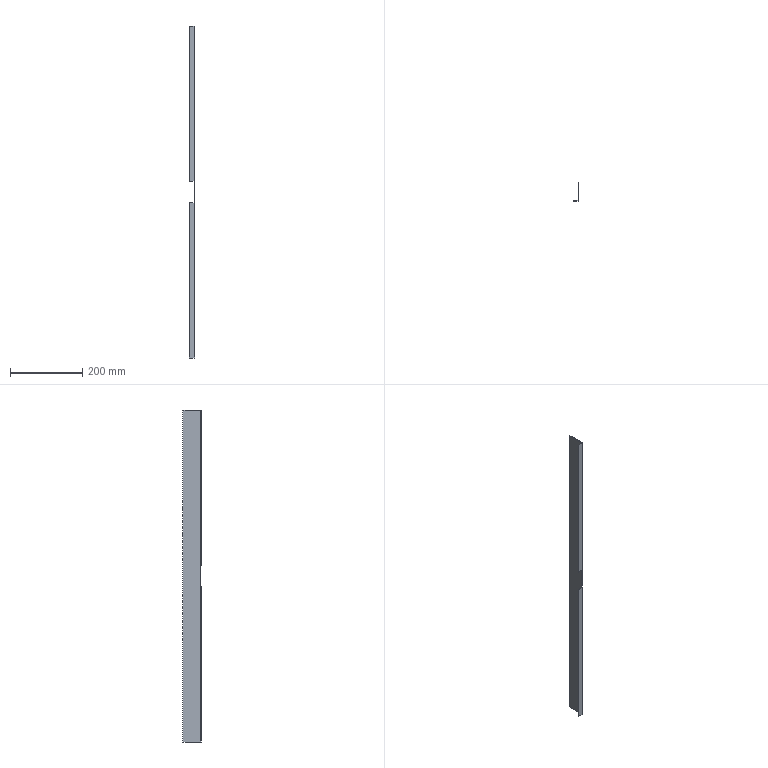Component | SolidWorks | UpperCrossbarRear400AType40001100-1 | 1 solid | 24 faces | box 16 x 50 x 920 mm | volume 86681 mm3 | plane 20 | cylinder 4 | commonest cylinder face diameters 4.473 x2 1.473 x2
STEP:
#1=COLOUR_RGB('',0.7922,0.8196,0.9333);
#2=FILL_AREA_STYLE_COLOUR('',#1);
#3=FILL_AREA_STYLE('',(#2));
#4=SURFACE_STYLE_FILL_AREA(#3);
#5=SURFACE_SIDE_STYLE('',(#4));
#6=SURFACE_STYLE_USAGE(.BOTH.,#5);
#7=PRESENTATION_STYLE_ASSIGNMENT((#6));
#8=CARTESIAN_POINT('',(11.469,40.827,37.736));
#9=VERTEX_POINT('',#8);
#10=CARTESIAN_POINT('',(11.469,40.827,20.807));
#11=VERTEX_POINT('',#10);
#12=CARTESIAN_POINT('',(11.469,40.827,1.516));
#13=DIRECTION('',(0.,0.,-1.));
#14=VECTOR('',#13,39.37);
#15=LINE('',#12,#14);
#16=EDGE_CURVE('',#9,#11,#15,.T.);
#17=ORIENTED_EDGE('',*,*,#16,.T.);
#18=CARTESIAN_POINT('',(11.557,40.915,20.807));
#19=VERTEX_POINT('',#18);
#20=CARTESIAN_POINT('',(11.469,40.915,20.807));
#21=DIRECTION('',(-0.,-0.,1.));
#22=DIRECTION('',(-1.,0.,0.));
#23=AXIS2_PLACEMENT_3D('',#20,#21,#22);
#24=CIRCLE('',#23,0.08806);
#25=EDGE_CURVE('',#11,#19,#24,.T.);
#26=ORIENTED_EDGE('',*,*,#25,.T.);
#27=CARTESIAN_POINT('',(11.557,40.915,37.736));
#28=VERTEX_POINT('',#27);
#29=CARTESIAN_POINT('',(11.557,40.915,37.736));
#30=DIRECTION('',(0.,0.,-1.));
#31=VECTOR('',#30,39.37);
#32=LINE('',#29,#31);
#33=EDGE_CURVE('',#28,#19,#32,.T.);
#34=ORIENTED_EDGE('',*,*,#33,.F.);
#35=CARTESIAN_POINT('',(11.469,40.915,37.736));
#36=DIRECTION('',(-0.,-0.,1.));
#37=DIRECTION('',(1.,0.,0.));
#38=AXIS2_PLACEMENT_3D('',#35,#36,#37);
#39=CIRCLE('',#38,0.08806);
#40=EDGE_CURVE('',#9,#28,#39,.T.);
#41=ORIENTED_EDGE('',*,*,#40,.F.);
#42=EDGE_LOOP('',(#17,#26,#34,#41));
#43=FACE_OUTER_BOUND('',#42,.T.);
#44=CARTESIAN_POINT('',(11.469,40.915,37.736));
#45=DIRECTION('',(-0.,-0.,1.));
#46=DIRECTION('',(0.,-1.,0.));
#47=AXIS2_PLACEMENT_3D('',#44,#45,#46);
#48=CYLINDRICAL_SURFACE('',#47,0.08806);
#49=ADVANCED_FACE('',(#43),#48,.T.);
#50=CARTESIAN_POINT('',(11.557,40.915,18.445));
#51=VERTEX_POINT('',#50);
#52=CARTESIAN_POINT('',(11.557,40.915,1.516));
#53=VERTEX_POINT('',#52);
#54=CARTESIAN_POINT('',(11.557,40.915,37.736));
#55=DIRECTION('',(0.,0.,-1.));
#56=VECTOR('',#55,39.37);
#57=LINE('',#54,#56);
#58=EDGE_CURVE('',#51,#53,#57,.T.);
#59=ORIENTED_EDGE('',*,*,#58,.F.);
#60=CARTESIAN_POINT('',(11.469,40.827,18.445));
#61=VERTEX_POINT('',#60);
#62=CARTESIAN_POINT('',(11.469,40.915,18.445));
#63=DIRECTION('',(0.,0.,-1.));
#64=DIRECTION('',(1.,0.,0.));
#65=AXIS2_PLACEMENT_3D('',#62,#63,#64);
#66=CIRCLE('',#65,0.08806);
#67=EDGE_CURVE('',#51,#61,#66,.T.);
#68=ORIENTED_EDGE('',*,*,#67,.T.);
#69=CARTESIAN_POINT('',(11.469,40.827,1.516));
#70=VERTEX_POINT('',#69);
#71=CARTESIAN_POINT('',(11.469,40.827,1.516));
#72=DIRECTION('',(0.,0.,-1.));
#73=VECTOR('',#72,39.37);
#74=LINE('',#71,#73);
#75=EDGE_CURVE('',#61,#70,#74,.T.);
#76=ORIENTED_EDGE('',*,*,#75,.T.);
#77=CARTESIAN_POINT('',(11.469,40.915,1.516));
#78=DIRECTION('',(0.,0.,-1.));
#79=DIRECTION('',(1.,0.,0.));
#80=AXIS2_PLACEMENT_3D('',#77,#78,#79);
#81=CIRCLE('',#80,0.08806);
#82=EDGE_CURVE('',#53,#70,#81,.T.);
#83=ORIENTED_EDGE('',*,*,#82,.F.);
#84=EDGE_LOOP('',(#59,#68,#76,#83));
#85=FACE_OUTER_BOUND('',#84,.T.);
#86=CARTESIAN_POINT('',(11.469,40.915,37.736));
#87=DIRECTION('',(-0.,-0.,1.));
#88=DIRECTION('',(0.,-1.,0.));
#89=AXIS2_PLACEMENT_3D('',#86,#87,#88);
#90=CYLINDRICAL_SURFACE('',#89,0.08806);
#91=ADVANCED_FACE('',(#85),#90,.T.);
#92=CARTESIAN_POINT('',(11.469,40.886,20.807));
#93=VERTEX_POINT('',#92);
#94=CARTESIAN_POINT('',(11.498,40.915,20.807));
#95=VERTEX_POINT('',#94);
#96=CARTESIAN_POINT('',(11.469,40.915,20.807));
#97=DIRECTION('',(-0.,-0.,1.));
#98=DIRECTION('',(1.,0.,0.));
#99=AXIS2_PLACEMENT_3D('',#96,#97,#98);
#100=CIRCLE('',#99,0.029);
#101=EDGE_CURVE('',#93,#95,#100,.T.);
#102=ORIENTED_EDGE('',*,*,#101,.F.);
#103=CARTESIAN_POINT('',(11.469,40.886,37.736));
#104=VERTEX_POINT('',#103);
#105=CARTESIAN_POINT('',(11.469,40.886,1.516));
#106=DIRECTION('',(-0.,-0.,1.));
#107=VECTOR('',#106,39.37);
#108=LINE('',#105,#107);
#109=EDGE_CURVE('',#93,#104,#108,.T.);
#110=ORIENTED_EDGE('',*,*,#109,.T.);
#111=CARTESIAN_POINT('',(11.498,40.915,37.736));
#112=VERTEX_POINT('',#111);
#113=CARTESIAN_POINT('',(11.469,40.915,37.736));
#114=DIRECTION('',(-0.,-0.,1.));
#115=DIRECTION('',(1.,0.,0.));
#116=AXIS2_PLACEMENT_3D('',#113,#114,#115);
#117=CIRCLE('',#116,0.029);
#118=EDGE_CURVE('',#104,#112,#117,.T.);
#119=ORIENTED_EDGE('',*,*,#118,.T.);
#120=CARTESIAN_POINT('',(11.498,40.915,37.736));
#121=DIRECTION('',(0.,0.,-1.));
#122=VECTOR('',#121,39.37);
#123=LINE('',#120,#122);
#124=EDGE_CURVE('',#112,#95,#123,.T.);
#125=ORIENTED_EDGE('',*,*,#124,.T.);
#126=EDGE_LOOP('',(#102,#110,#119,#125));
#127=FACE_OUTER_BOUND('',#126,.T.);
#128=CARTESIAN_POINT('',(11.469,40.915,37.736));
#129=DIRECTION('',(-0.,-0.,1.));
#130=DIRECTION('',(0.,-1.,0.));
#131=AXIS2_PLACEMENT_3D('',#128,#129,#130);
#132=CYLINDRICAL_SURFACE('',#131,0.029);
#133=ADVANCED_FACE('',(#127),#132,.F.);
#134=CARTESIAN_POINT('',(11.498,40.915,18.445));
#135=VERTEX_POINT('',#134);
#136=CARTESIAN_POINT('',(11.469,40.886,18.445));
#137=VERTEX_POINT('',#136);
#138=CARTESIAN_POINT('',(11.469,40.915,18.445));
#139=DIRECTION('',(0.,0.,-1.));
#140=DIRECTION('',(1.,0.,0.));
#141=AXIS2_PLACEMENT_3D('',#138,#139,#140);
#142=CIRCLE('',#141,0.029);
#143=EDGE_CURVE('',#135,#137,#142,.T.);
#144=ORIENTED_EDGE('',*,*,#143,.F.);
#145=CARTESIAN_POINT('',(11.498,40.915,1.516));
#146=VERTEX_POINT('',#145);
#147=CARTESIAN_POINT('',(11.498,40.915,37.736));
#148=DIRECTION('',(0.,0.,-1.));
#149=VECTOR('',#148,39.37);
#150=LINE('',#147,#149);
#151=EDGE_CURVE('',#135,#146,#150,.T.);
#152=ORIENTED_EDGE('',*,*,#151,.T.);
#153=CARTESIAN_POINT('',(11.469,40.886,1.516));
#154=VERTEX_POINT('',#153);
#155=CARTESIAN_POINT('',(11.469,40.915,1.516));
#156=DIRECTION('',(0.,0.,-1.));
#157=DIRECTION('',(1.,0.,0.));
#158=AXIS2_PLACEMENT_3D('',#155,#156,#157);
#159=CIRCLE('',#158,0.029);
#160=EDGE_CURVE('',#146,#154,#159,.T.);
#161=ORIENTED_EDGE('',*,*,#160,.T.);
#162=CARTESIAN_POINT('',(11.469,40.886,1.516));
#163=DIRECTION('',(-0.,-0.,1.));
#164=VECTOR('',#163,39.37);
#165=LINE('',#162,#164);
#166=EDGE_CURVE('',#154,#137,#165,.T.);
#167=ORIENTED_EDGE('',*,*,#166,.T.);
#168=EDGE_LOOP('',(#144,#152,#161,#167));
#169=FACE_OUTER_BOUND('',#168,.T.);
#170=CARTESIAN_POINT('',(11.469,40.915,37.736));
#171=DIRECTION('',(-0.,-0.,1.));
#172=DIRECTION('',(0.,-1.,0.));
#173=AXIS2_PLACEMENT_3D('',#170,#171,#172);
#174=CYLINDRICAL_SURFACE('',#173,0.029);
#175=ADVANCED_FACE('',(#169),#174,.F.);
#176=CARTESIAN_POINT('',(10.927,40.827,20.807));
#177=VERTEX_POINT('',#176);
#178=CARTESIAN_POINT('',(10.927,40.827,20.807));
#179=DIRECTION('',(1.,0.,0.));
#180=VECTOR('',#179,39.37);
#181=LINE('',#178,#180);
#182=EDGE_CURVE('',#177,#11,#181,.T.);
#183=ORIENTED_EDGE('',*,*,#182,.T.);
#184=ORIENTED_EDGE('',*,*,#16,.F.);
#185=CARTESIAN_POINT('',(10.927,40.827,37.736));
#186=VERTEX_POINT('',#185);
#187=CARTESIAN_POINT('',(10.927,40.827,37.736));
#188=DIRECTION('',(-1.,-0.,-0.));
#189=VECTOR('',#188,39.37);
#190=LINE('',#187,#189);
#191=EDGE_CURVE('',#9,#186,#190,.T.);
#192=ORIENTED_EDGE('',*,*,#191,.T.);
#193=CARTESIAN_POINT('',(10.927,40.827,1.516));
#194=DIRECTION('',(0.,0.,-1.));
#195=VECTOR('',#194,39.37);
#196=LINE('',#193,#195);
#197=EDGE_CURVE('',#186,#177,#196,.T.);
#198=ORIENTED_EDGE('',*,*,#197,.T.);
#199=EDGE_LOOP('',(#183,#184,#192,#198));
#200=FACE_OUTER_BOUND('',#199,.T.);
#201=CARTESIAN_POINT('',(10.927,40.827,1.516));
#202=DIRECTION('',(-0.,1.,0.));
#203=DIRECTION('',(-1.,-0.,-0.));
#204=AXIS2_PLACEMENT_3D('',#201,#202,#203);
#205=PLANE('',#204);
#206=ADVANCED_FACE('',(#200),#205,.F.);
#207=CARTESIAN_POINT('',(10.927,40.827,18.445));
#208=VERTEX_POINT('',#207);
#209=CARTESIAN_POINT('',(10.927,40.827,18.445));
#210=DIRECTION('',(1.,0.,0.));
#211=VECTOR('',#210,39.37);
#212=LINE('',#209,#211);
#213=EDGE_CURVE('',#208,#61,#212,.T.);
#214=ORIENTED_EDGE('',*,*,#213,.F.);
#215=CARTESIAN_POINT('',(10.927,40.827,1.516));
#216=VERTEX_POINT('',#215);
#217=CARTESIAN_POINT('',(10.927,40.827,1.516));
#218=DIRECTION('',(0.,0.,-1.));
#219=VECTOR('',#218,39.37);
#220=LINE('',#217,#219);
#221=EDGE_CURVE('',#208,#216,#220,.T.);
#222=ORIENTED_EDGE('',*,*,#221,.T.);
#223=CARTESIAN_POINT('',(10.927,40.827,1.516));
#224=DIRECTION('',(1.,0.,0.));
#225=VECTOR('',#224,39.37);
#226=LINE('',#223,#225);
#227=EDGE_CURVE('',#216,#70,#226,.T.);
#228=ORIENTED_EDGE('',*,*,#227,.T.);
#229=ORIENTED_EDGE('',*,*,#75,.F.);
#230=EDGE_LOOP('',(#214,#222,#228,#229));
#231=FACE_OUTER_BOUND('',#230,.T.);
#232=CARTESIAN_POINT('',(10.927,40.827,1.516));
#233=DIRECTION('',(-0.,1.,0.));
#234=DIRECTION('',(-1.,-0.,-0.));
#235=AXIS2_PLACEMENT_3D('',#232,#233,#234);
#236=PLANE('',#235);
#237=ADVANCED_FACE('',(#231),#236,.F.);
#238=ORIENTED_EDGE('',*,*,#109,.F.);
#239=CARTESIAN_POINT('',(10.927,40.886,20.807));
#240=VERTEX_POINT('',#239);
#241=CARTESIAN_POINT('',(10.927,40.886,20.807));
#242=DIRECTION('',(1.,0.,0.));
#243=VECTOR('',#242,39.37);
#244=LINE('',#241,#243);
#245=EDGE_CURVE('',#240,#93,#244,.T.);
#246=ORIENTED_EDGE('',*,*,#245,.F.);
#247=CARTESIAN_POINT('',(10.927,40.886,37.736));
#248=VERTEX_POINT('',#247);
#249=CARTESIAN_POINT('',(10.927,40.886,1.516));
#250=DIRECTION('',(0.,0.,-1.));
#251=VECTOR('',#250,39.37);
#252=LINE('',#249,#251);
#253=EDGE_CURVE('',#248,#240,#252,.T.);
#254=ORIENTED_EDGE('',*,*,#253,.F.);
#255=CARTESIAN_POINT('',(10.927,40.886,37.736));
#256=DIRECTION('',(-1.,-0.,-0.));
#257=VECTOR('',#256,39.37);
#258=LINE('',#255,#257);
#259=EDGE_CURVE('',#104,#248,#258,.T.);
#260=ORIENTED_EDGE('',*,*,#259,.F.);
#261=EDGE_LOOP('',(#238,#246,#254,#260));
#262=FACE_OUTER_BOUND('',#261,.T.);
#263=CARTESIAN_POINT('',(10.927,40.886,1.516));
#264=DIRECTION('',(-0.,1.,0.));
#265=DIRECTION('',(-1.,-0.,-0.));
#266=AXIS2_PLACEMENT_3D('',#263,#264,#265);
#267=PLANE('',#266);
#268=ADVANCED_FACE('',(#262),#267,.T.);
#269=CARTESIAN_POINT('',(10.927,40.886,18.445));
#270=VERTEX_POINT('',#269);
#271=CARTESIAN_POINT('',(10.927,40.886,1.516));
#272=VERTEX_POINT('',#271);
#273=CARTESIAN_POINT('',(10.927,40.886,1.516));
#274=DIRECTION('',(0.,0.,-1.));
#275=VECTOR('',#274,39.37);
#276=LINE('',#273,#275);
#277=EDGE_CURVE('',#270,#272,#276,.T.);
#278=ORIENTED_EDGE('',*,*,#277,.F.);
#279=CARTESIAN_POINT('',(10.927,40.886,18.445));
#280=DIRECTION('',(1.,0.,0.));
#281=VECTOR('',#280,39.37);
#282=LINE('',#279,#281);
#283=EDGE_CURVE('',#270,#137,#282,.T.);
#284=ORIENTED_EDGE('',*,*,#283,.T.);
#285=ORIENTED_EDGE('',*,*,#166,.F.);
#286=CARTESIAN_POINT('',(11.498,40.886,1.516));
#287=DIRECTION('',(1.,0.,0.));
#288=VECTOR('',#287,39.37);
#289=LINE('',#286,#288);
#290=EDGE_CURVE('',#272,#154,#289,.T.);
#291=ORIENTED_EDGE('',*,*,#290,.F.);
#292=EDGE_LOOP('',(#278,#284,#285,#291));
#293=FACE_OUTER_BOUND('',#292,.T.);
#294=CARTESIAN_POINT('',(10.927,40.886,1.516));
#295=DIRECTION('',(-0.,1.,0.));
#296=DIRECTION('',(-1.,-0.,-0.));
#297=AXIS2_PLACEMENT_3D('',#294,#295,#296);
#298=PLANE('',#297);
#299=ADVANCED_FACE('',(#293),#298,.T.);
#300=CARTESIAN_POINT('',(10.927,40.827,20.807));
#301=DIRECTION('',(-0.,1.,0.));
#302=VECTOR('',#301,39.37);
#303=LINE('',#300,#302);
#304=EDGE_CURVE('',#177,#240,#303,.T.);
#305=ORIENTED_EDGE('',*,*,#304,.F.);
#306=ORIENTED_EDGE('',*,*,#197,.F.);
#307=CARTESIAN_POINT('',(10.927,40.827,37.736));
#308=DIRECTION('',(-0.,1.,0.));
#309=VECTOR('',#308,39.37);
#310=LINE('',#307,#309);
#311=EDGE_CURVE('',#186,#248,#310,.T.);
#312=ORIENTED_EDGE('',*,*,#311,.T.);
#313=ORIENTED_EDGE('',*,*,#253,.T.);
#314=EDGE_LOOP('',(#305,#306,#312,#313));
#315=FACE_OUTER_BOUND('',#314,.T.);
#316=CARTESIAN_POINT('',(10.927,40.827,1.516));
#317=DIRECTION('',(1.,0.,0.));
#318=DIRECTION('',(-0.,1.,0.));
#319=AXIS2_PLACEMENT_3D('',#316,#317,#318);
#320=PLANE('',#319);
#321=ADVANCED_FACE('',(#315),#320,.F.);
#322=CARTESIAN_POINT('',(10.927,40.827,18.445));
#323=DIRECTION('',(-0.,1.,0.));
#324=VECTOR('',#323,39.37);
#325=LINE('',#322,#324);
#326=EDGE_CURVE('',#208,#270,#325,.T.);
#327=ORIENTED_EDGE('',*,*,#326,.T.);
#328=ORIENTED_EDGE('',*,*,#277,.T.);
#329=CARTESIAN_POINT('',(10.927,40.827,1.516));
#330=DIRECTION('',(-0.,1.,0.));
#331=VECTOR('',#330,39.37);
#332=LINE('',#329,#331);
#333=EDGE_CURVE('',#216,#272,#332,.T.);
#334=ORIENTED_EDGE('',*,*,#333,.F.);
#335=ORIENTED_EDGE('',*,*,#221,.F.);
#336=EDGE_LOOP('',(#327,#328,#334,#335));
#337=FACE_OUTER_BOUND('',#336,.T.);
#338=CARTESIAN_POINT('',(10.927,40.827,1.516));
#339=DIRECTION('',(1.,0.,0.));
#340=DIRECTION('',(-0.,1.,0.));
#341=AXIS2_PLACEMENT_3D('',#338,#339,#340);
#342=PLANE('',#341);
#343=ADVANCED_FACE('',(#337),#342,.F.);
#344=CARTESIAN_POINT('',(11.498,42.795,37.736));
#345=VERTEX_POINT('',#344);
#346=CARTESIAN_POINT('',(11.498,40.827,37.736));
#347=DIRECTION('',(-0.,1.,0.));
#348=VECTOR('',#347,39.37);
#349=LINE('',#346,#348);
#350=EDGE_CURVE('',#112,#345,#349,.T.);
#351=ORIENTED_EDGE('',*,*,#350,.F.);
#352=CARTESIAN_POINT('',(11.498,40.915,37.736));
#353=DIRECTION('',(1.,0.,0.));
#354=VECTOR('',#353,39.37);
#355=LINE('',#352,#354);
#356=EDGE_CURVE('',#112,#28,#355,.T.);
#357=ORIENTED_EDGE('',*,*,#356,.T.);
#358=CARTESIAN_POINT('',(11.557,42.795,37.736));
#359=VERTEX_POINT('',#358);
#360=CARTESIAN_POINT('',(11.557,40.827,37.736));
#361=DIRECTION('',(-0.,1.,0.));
#362=VECTOR('',#361,39.37);
#363=LINE('',#360,#362);
#364=EDGE_CURVE('',#28,#359,#363,.T.);
#365=ORIENTED_EDGE('',*,*,#364,.T.);
#366=CARTESIAN_POINT('',(11.557,42.795,37.736));
#367=DIRECTION('',(-1.,-0.,-0.));
#368=VECTOR('',#367,39.37);
#369=LINE('',#366,#368);
#370=EDGE_CURVE('',#359,#345,#369,.T.);
#371=ORIENTED_EDGE('',*,*,#370,.T.);
#372=EDGE_LOOP('',(#351,#357,#365,#371));
#373=FACE_OUTER_BOUND('',#372,.T.);
#374=CARTESIAN_POINT('',(11.557,40.827,37.736));
#375=DIRECTION('',(-0.,-0.,1.));
#376=DIRECTION('',(1.,0.,0.));
#377=AXIS2_PLACEMENT_3D('',#374,#375,#376);
#378=PLANE('',#377);
#379=ADVANCED_FACE('',(#373),#378,.T.);
#380=ORIENTED_EDGE('',*,*,#33,.T.);
#381=CARTESIAN_POINT('',(11.557,40.915,37.736));
#382=DIRECTION('',(0.,0.,-1.));
#383=VECTOR('',#382,39.37);
#384=LINE('',#381,#383);
#385=EDGE_CURVE('',#19,#51,#384,.T.);
#386=ORIENTED_EDGE('',*,*,#385,.T.);
#387=ORIENTED_EDGE('',*,*,#58,.T.);
#388=CARTESIAN_POINT('',(11.557,42.795,1.516));
#389=VERTEX_POINT('',#388);
#390=CARTESIAN_POINT('',(11.557,40.827,1.516));
#391=DIRECTION('',(0.,-1.,-0.));
#392=VECTOR('',#391,39.37);
#393=LINE('',#390,#392);
#394=EDGE_CURVE('',#389,#53,#393,.T.);
#395=ORIENTED_EDGE('',*,*,#394,.F.);
#396=CARTESIAN_POINT('',(11.557,42.795,37.736));
#397=DIRECTION('',(0.,0.,-1.));
#398=VECTOR('',#397,39.37);
#399=LINE('',#396,#398);
#400=EDGE_CURVE('',#359,#389,#399,.T.);
#401=ORIENTED_EDGE('',*,*,#400,.F.);
#402=ORIENTED_EDGE('',*,*,#364,.F.);
#403=EDGE_LOOP('',(#380,#386,#387,#395,#401,#402));
#404=FACE_OUTER_BOUND('',#403,.T.);
#405=CARTESIAN_POINT('',(11.557,42.795,37.736));
#406=DIRECTION('',(-1.,-0.,-0.));
#407=DIRECTION('',(-0.,-0.,1.));
#408=AXIS2_PLACEMENT_3D('',#405,#406,#407);
#409=PLANE('',#408);
#410=ADVANCED_FACE('',(#404),#409,.F.);
#411=CARTESIAN_POINT('',(11.498,42.795,1.516));
#412=VERTEX_POINT('',#411);
#413=CARTESIAN_POINT('',(11.498,40.827,1.516));
#414=DIRECTION('',(0.,-1.,-0.));
#415=VECTOR('',#414,39.37);
#416=LINE('',#413,#415);
#417=EDGE_CURVE('',#412,#146,#416,.T.);
#418=ORIENTED_EDGE('',*,*,#417,.T.);
#419=ORIENTED_EDGE('',*,*,#151,.F.);
#420=CARTESIAN_POINT('',(11.498,40.915,37.736));
#421=DIRECTION('',(0.,0.,-1.));
#422=VECTOR('',#421,39.37);
#423=LINE('',#420,#422);
#424=EDGE_CURVE('',#95,#135,#423,.T.);
#425=ORIENTED_EDGE('',*,*,#424,.F.);
#426=ORIENTED_EDGE('',*,*,#124,.F.);
#427=ORIENTED_EDGE('',*,*,#350,.T.);
#428=CARTESIAN_POINT('',(11.498,42.795,37.736));
#429=DIRECTION('',(0.,0.,-1.));
#430=VECTOR('',#429,39.37);
#431=LINE('',#428,#430);
#432=EDGE_CURVE('',#345,#412,#431,.T.);
#433=ORIENTED_EDGE('',*,*,#432,.T.);
#434=EDGE_LOOP('',(#418,#419,#425,#426,#427,#433));
#435=FACE_OUTER_BOUND('',#434,.T.);
#436=CARTESIAN_POINT('',(11.498,42.795,37.736));
#437=DIRECTION('',(-1.,-0.,-0.));
#438=DIRECTION('',(-0.,-0.,1.));
#439=AXIS2_PLACEMENT_3D('',#436,#437,#438);
#440=PLANE('',#439);
#441=ADVANCED_FACE('',(#435),#440,.T.);
#442=CARTESIAN_POINT('',(11.498,40.915,1.516));
#443=DIRECTION('',(1.,0.,0.));
#444=VECTOR('',#443,39.37);
#445=LINE('',#442,#444);
#446=EDGE_CURVE('',#146,#53,#445,.T.);
#447=ORIENTED_EDGE('',*,*,#446,.F.);
#448=ORIENTED_EDGE('',*,*,#417,.F.);
#449=CARTESIAN_POINT('',(11.557,42.795,1.516));
#450=DIRECTION('',(-1.,-0.,-0.));
#451=VECTOR('',#450,39.37);
#452=LINE('',#449,#451);
#453=EDGE_CURVE('',#389,#412,#452,.T.);
#454=ORIENTED_EDGE('',*,*,#453,.F.);
#455=ORIENTED_EDGE('',*,*,#394,.T.);
#456=EDGE_LOOP('',(#447,#448,#454,#455));
#457=FACE_OUTER_BOUND('',#456,.T.);
#458=CARTESIAN_POINT('',(11.557,40.827,1.516));
#459=DIRECTION('',(0.,0.,-1.));
#460=DIRECTION('',(-1.,-0.,-0.));
#461=AXIS2_PLACEMENT_3D('',#458,#459,#460);
#462=PLANE('',#461);
#463=ADVANCED_FACE('',(#457),#462,.T.);
#464=ORIENTED_EDGE('',*,*,#432,.F.);
#465=ORIENTED_EDGE('',*,*,#370,.F.);
#466=ORIENTED_EDGE('',*,*,#400,.T.);
#467=ORIENTED_EDGE('',*,*,#453,.T.);
#468=EDGE_LOOP('',(#464,#465,#466,#467));
#469=FACE_OUTER_BOUND('',#468,.T.);
#470=CARTESIAN_POINT('',(11.557,42.795,37.736));
#471=DIRECTION('',(-0.,1.,0.));
#472=DIRECTION('',(0.,0.,-1.));
#473=AXIS2_PLACEMENT_3D('',#470,#471,#472);
#474=PLANE('',#473);
#475=ADVANCED_FACE('',(#469),#474,.T.);
#476=CARTESIAN_POINT('',(11.469,40.827,1.516));
#477=DIRECTION('',(0.,-1.,-0.));
#478=VECTOR('',#477,39.37);
#479=LINE('',#476,#478);
#480=EDGE_CURVE('',#154,#70,#479,.T.);
#481=ORIENTED_EDGE('',*,*,#480,.F.);
#482=ORIENTED_EDGE('',*,*,#160,.F.);
#483=ORIENTED_EDGE('',*,*,#446,.T.);
#484=ORIENTED_EDGE('',*,*,#82,.T.);
#485=EDGE_LOOP('',(#481,#482,#483,#484));
#486=FACE_OUTER_BOUND('',#485,.T.);
#487=CARTESIAN_POINT('',(11.469,40.915,1.516));
#488=DIRECTION('',(0.,0.,-1.));
#489=DIRECTION('',(-1.,0.,-0.));
#490=AXIS2_PLACEMENT_3D('',#487,#488,#489);
#491=PLANE('',#490);
#492=ADVANCED_FACE('',(#486),#491,.T.);
#493=ORIENTED_EDGE('',*,*,#118,.F.);
#494=CARTESIAN_POINT('',(11.469,40.886,37.736));
#495=DIRECTION('',(0.,-1.,-0.));
#496=VECTOR('',#495,39.37);
#497=LINE('',#494,#496);
#498=EDGE_CURVE('',#104,#9,#497,.T.);
#499=ORIENTED_EDGE('',*,*,#498,.T.);
#500=ORIENTED_EDGE('',*,*,#40,.T.);
#501=ORIENTED_EDGE('',*,*,#356,.F.);
#502=EDGE_LOOP('',(#493,#499,#500,#501));
#503=FACE_OUTER_BOUND('',#502,.T.);
#504=CARTESIAN_POINT('',(11.469,40.915,37.736));
#505=DIRECTION('',(0.,0.,-1.));
#506=DIRECTION('',(-1.,0.,-0.));
#507=AXIS2_PLACEMENT_3D('',#504,#505,#506);
#508=PLANE('',#507);
#509=ADVANCED_FACE('',(#503),#508,.F.);
#510=ORIENTED_EDGE('',*,*,#480,.T.);
#511=ORIENTED_EDGE('',*,*,#227,.F.);
#512=ORIENTED_EDGE('',*,*,#333,.T.);
#513=ORIENTED_EDGE('',*,*,#290,.T.);
#514=EDGE_LOOP('',(#510,#511,#512,#513));
#515=FACE_OUTER_BOUND('',#514,.T.);
#516=CARTESIAN_POINT('',(11.498,40.827,1.516));
#517=DIRECTION('',(-0.,-0.,1.));
#518=DIRECTION('',(-0.,1.,0.));
#519=AXIS2_PLACEMENT_3D('',#516,#517,#518);
#520=PLANE('',#519);
#521=ADVANCED_FACE('',(#515),#520,.F.);
#522=ORIENTED_EDGE('',*,*,#498,.F.);
#523=ORIENTED_EDGE('',*,*,#259,.T.);
#524=ORIENTED_EDGE('',*,*,#311,.F.);
#525=ORIENTED_EDGE('',*,*,#191,.F.);
#526=EDGE_LOOP('',(#522,#523,#524,#525));
#527=FACE_OUTER_BOUND('',#526,.T.);
#528=CARTESIAN_POINT('',(10.927,40.827,37.736));
#529=DIRECTION('',(0.,0.,-1.));
#530=DIRECTION('',(0.,-1.,-0.));
#531=AXIS2_PLACEMENT_3D('',#528,#529,#530);
#532=PLANE('',#531);
#533=ADVANCED_FACE('',(#527),#532,.F.);
#534=CARTESIAN_POINT('',(11.469,40.827,20.807));
#535=DIRECTION('',(-0.,1.,0.));
#536=VECTOR('',#535,39.37);
#537=LINE('',#534,#536);
#538=EDGE_CURVE('',#11,#93,#537,.T.);
#539=ORIENTED_EDGE('',*,*,#538,.F.);
#540=ORIENTED_EDGE('',*,*,#182,.F.);
#541=ORIENTED_EDGE('',*,*,#304,.T.);
#542=ORIENTED_EDGE('',*,*,#245,.T.);
#543=EDGE_LOOP('',(#539,#540,#541,#542));
#544=FACE_OUTER_BOUND('',#543,.T.);
#545=CARTESIAN_POINT('',(10.927,40.827,20.807));
#546=DIRECTION('',(-0.,-0.,1.));
#547=DIRECTION('',(1.,0.,0.));
#548=AXIS2_PLACEMENT_3D('',#545,#546,#547);
#549=PLANE('',#548);
#550=ADVANCED_FACE('',(#544),#549,.F.);
#551=ORIENTED_EDGE('',*,*,#213,.T.);
#552=CARTESIAN_POINT('',(11.469,40.827,18.445));
#553=DIRECTION('',(-0.,1.,0.));
#554=VECTOR('',#553,39.37);
#555=LINE('',#552,#554);
#556=EDGE_CURVE('',#61,#137,#555,.T.);
#557=ORIENTED_EDGE('',*,*,#556,.T.);
#558=ORIENTED_EDGE('',*,*,#283,.F.);
#559=ORIENTED_EDGE('',*,*,#326,.F.);
#560=EDGE_LOOP('',(#551,#557,#558,#559));
#561=FACE_OUTER_BOUND('',#560,.T.);
#562=CARTESIAN_POINT('',(10.927,40.827,18.445));
#563=DIRECTION('',(-0.,-0.,1.));
#564=DIRECTION('',(1.,0.,0.));
#565=AXIS2_PLACEMENT_3D('',#562,#563,#564);
#566=PLANE('',#565);
#567=ADVANCED_FACE('',(#561),#566,.T.);
#568=ORIENTED_EDGE('',*,*,#25,.F.);
#569=ORIENTED_EDGE('',*,*,#538,.T.);
#570=ORIENTED_EDGE('',*,*,#101,.T.);
#571=CARTESIAN_POINT('',(11.498,40.915,20.807));
#572=DIRECTION('',(1.,0.,0.));
#573=VECTOR('',#572,39.37);
#574=LINE('',#571,#573);
#575=EDGE_CURVE('',#95,#19,#574,.T.);
#576=ORIENTED_EDGE('',*,*,#575,.T.);
#577=EDGE_LOOP('',(#568,#569,#570,#576));
#578=FACE_OUTER_BOUND('',#577,.T.);
#579=CARTESIAN_POINT('',(11.469,40.915,20.807));
#580=DIRECTION('',(-0.,-0.,1.));
#581=DIRECTION('',(1.,0.,0.));
#582=AXIS2_PLACEMENT_3D('',#579,#580,#581);
#583=PLANE('',#582);
#584=ADVANCED_FACE('',(#578),#583,.F.);
#585=ORIENTED_EDGE('',*,*,#556,.F.);
#586=ORIENTED_EDGE('',*,*,#67,.F.);
#587=CARTESIAN_POINT('',(11.498,40.915,18.445));
#588=DIRECTION('',(1.,0.,0.));
#589=VECTOR('',#588,39.37);
#590=LINE('',#587,#589);
#591=EDGE_CURVE('',#135,#51,#590,.T.);
#592=ORIENTED_EDGE('',*,*,#591,.F.);
#593=ORIENTED_EDGE('',*,*,#143,.T.);
#594=EDGE_LOOP('',(#585,#586,#592,#593));
#595=FACE_OUTER_BOUND('',#594,.T.);
#596=CARTESIAN_POINT('',(11.469,40.915,18.445));
#597=DIRECTION('',(0.,0.,-1.));
#598=DIRECTION('',(-1.,-0.,-0.));
#599=AXIS2_PLACEMENT_3D('',#596,#597,#598);
#600=PLANE('',#599);
#601=ADVANCED_FACE('',(#595),#600,.F.);
#602=ORIENTED_EDGE('',*,*,#575,.F.);
#603=ORIENTED_EDGE('',*,*,#424,.T.);
#604=ORIENTED_EDGE('',*,*,#591,.T.);
#605=ORIENTED_EDGE('',*,*,#385,.F.);
#606=EDGE_LOOP('',(#602,#603,#604,#605));
#607=FACE_OUTER_BOUND('',#606,.T.);
#608=CARTESIAN_POINT('',(11.498,40.915,19.626));
#609=DIRECTION('',(-0.,1.,0.));
#610=DIRECTION('',(-0.,-0.,1.));
#611=AXIS2_PLACEMENT_3D('',#608,#609,#610);
#612=PLANE('',#611);
#613=ADVANCED_FACE('',(#607),#612,.F.);
#614=CLOSED_SHELL('',(#49,#91,#133,#175,#206,#237,#268,#299,#321,#343,#379,#410,#441,#463,#475,#492,#509,#521,#533,#550,#567,#584,#601,#613));
#615=MANIFOLD_SOLID_BREP('',#614);
#616=STYLED_ITEM('',(#7),#615);
#617=(LENGTH_UNIT()NAMED_UNIT(*)SI_UNIT($,.METRE.));
#618=LENGTH_MEASURE_WITH_UNIT(LENGTH_MEASURE(0.0254),#617);
#619=DIMENSIONAL_EXPONENTS(1.,0.,0.,0.,0.,0.,0.);
#620=(CONVERSION_BASED_UNIT('',#618)LENGTH_UNIT()NAMED_UNIT(#619));
#621=UNCERTAINTY_MEASURE_WITH_UNIT(LENGTH_MEASURE(0.00001),#620,'','');
#622=(NAMED_UNIT(*)PLANE_ANGLE_UNIT()SI_UNIT($,.RADIAN.));
#623=(NAMED_UNIT(*)SI_UNIT($,.STERADIAN.)SOLID_ANGLE_UNIT());
#624=(GEOMETRIC_REPRESENTATION_CONTEXT(3)GLOBAL_UNCERTAINTY_ASSIGNED_CONTEXT((#621))GLOBAL_UNIT_ASSIGNED_CONTEXT((#620,#622,#623))REPRESENTATION_CONTEXT('',''));
#625=MECHANICAL_DESIGN_GEOMETRIC_PRESENTATION_REPRESENTATION('',(#616),#624);
#626=PRESENTATION_LAYER_ASSIGNMENT('','',(#616));
#627=CARTESIAN_POINT('',(0.,0.,0.));
#628=DIRECTION('',(0.,0.,1.));
#629=DIRECTION('',(1.,0.,0.));
#630=AXIS2_PLACEMENT_3D('',#627,#628,#629);
#631=(LENGTH_UNIT()NAMED_UNIT(*)SI_UNIT($,.METRE.));
#632=LENGTH_MEASURE_WITH_UNIT(LENGTH_MEASURE(0.0254),#631);
#633=DIMENSIONAL_EXPONENTS(1.,0.,0.,0.,0.,0.,0.);
#634=(CONVERSION_BASED_UNIT('',#632)LENGTH_UNIT()NAMED_UNIT(#633));
#635=UNCERTAINTY_MEASURE_WITH_UNIT(LENGTH_MEASURE(0.00001),#634,'','');
#636=(NAMED_UNIT(*)PLANE_ANGLE_UNIT()SI_UNIT($,.RADIAN.));
#637=(NAMED_UNIT(*)SI_UNIT($,.STERADIAN.)SOLID_ANGLE_UNIT());
#638=(GEOMETRIC_REPRESENTATION_CONTEXT(3)GLOBAL_UNCERTAINTY_ASSIGNED_CONTEXT((#635))GLOBAL_UNIT_ASSIGNED_CONTEXT((#634,#636,#637))REPRESENTATION_CONTEXT('',''));
#639=ADVANCED_BREP_SHAPE_REPRESENTATION('',(#615,#630),#638);